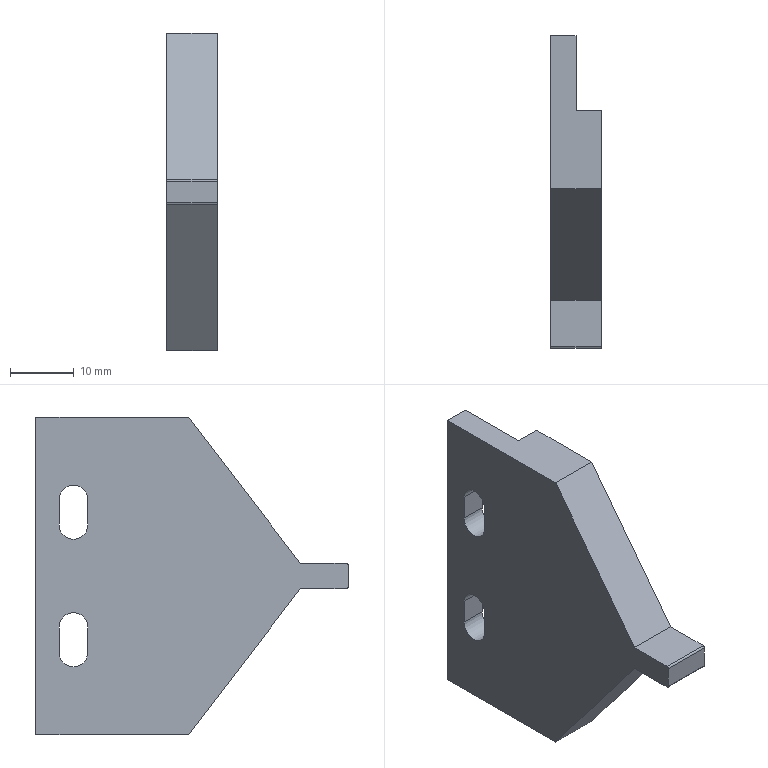Component | SolidWorks | WirePressingUnitPressingHead-2 | 1 solid | 24 faces | box 8 x 49 x 49.8 mm | volume 10945 mm3 | plane 16 | cylinder 8 | commonest cylinder face diameters 4.5 x6 0.6 x2
build123d program:
from build123d import *

# Parameters (mm, degrees)
BOSS_EXTRUDE1_DEPTH = 8
SKETCH2_W           = 49.8
SKETCH2_H           = 11.8
CUT_EXTRUDE1_DEPTH  = 4
SKETCH4_W           = 45.507
SKETCH4_H           = 8.951
BOSS_EXTRUDE2_DEPTH = 4
CUT_EXTRUDE3_DEPTH  = 10
FILLET1_R           = 0.3


with BuildPart() as part:
    # Sketch1 → Boss-Extrude1 (new body)
    with BuildSketch(Plane.XY):
        Polygon((2, 0), (2, 7.5), (24.9, 25), (24.9, 49), (-24.9, 49), (-24.9, 25), (-2, 7.5), (-2, 0), align=None)
    extrude(amount=BOSS_EXTRUDE1_DEPTH)

    # Sketch2 → Cut-Extrude1 (cut)
    with BuildSketch(Plane.XY.offset(8)):
        with Locations((0, 43.1)):
            Rectangle(SKETCH2_W, SKETCH2_H)
    extrude(amount=-CUT_EXTRUDE1_DEPTH, mode=Mode.SUBTRACT)

    # Sketch4 → Boss-Extrude2 (add)
    with BuildSketch(Plane(origin=(0, 0, 0), x_dir=(-1, 0, 0), z_dir=(0, 0, -1))):
        with Locations((-0.1161, 35.176)):
            Rectangle(SKETCH4_W, SKETCH4_H)
    extrude(amount=-BOSS_EXTRUDE2_DEPTH)

    # Sketch5 → Cut-Extrude3 (cut)
    with BuildSketch(Plane(origin=(0, 0, 0), x_dir=(-1, 0, 0), z_dir=(0, 0, -1))):
        with BuildLine():
            Line((-8, 40.85), (-12, 40.85))
            ThreePointArc((-12, 40.85), (-14.25, 43.1), (-12, 45.35))
            Line((-12, 45.35), (-8, 45.35))
            ThreePointArc((-8, 45.35), (-5.75, 43.1), (-8, 40.85))
        make_face()
        with BuildLine():
            Line((8, 45.35), (12, 45.35))
            ThreePointArc((12, 45.35), (14.25, 43.1), (12, 40.85))
            Line((12, 40.85), (8, 40.85))
            ThreePointArc((8, 40.85), (5.75, 43.1), (8, 45.35))
        make_face()
    extrude(amount=-CUT_EXTRUDE3_DEPTH, mode=Mode.SUBTRACT)

    # Fillet1
    fillet1_edges = [part.edges().sort_by_distance(p)[0] for p in [
        (-2, 0, 4),
        (2, 0, 4),
    ]]
    fillet(fillet1_edges, radius=FILLET1_R)


solid = part.part

# Placed as in the assembly
solid = solid.moved(Location((-17.235, -9.832, -145.015), (0, 90, 0)))
STEP:
#1=COLOUR_RGB('',0.7922,0.8196,0.9333);
#2=FILL_AREA_STYLE_COLOUR('',#1);
#3=FILL_AREA_STYLE('',(#2));
#4=SURFACE_STYLE_FILL_AREA(#3);
#5=SURFACE_SIDE_STYLE('',(#4));
#6=SURFACE_STYLE_USAGE(.BOTH.,#5);
#7=PRESENTATION_STYLE_ASSIGNMENT((#6));
#8=CARTESIAN_POINT('',(-0.5211,1.398,-5.237));
#9=VERTEX_POINT('',#8);
#10=CARTESIAN_POINT('',(-0.5211,1.31,-5.148));
#11=VERTEX_POINT('',#10);
#12=CARTESIAN_POINT('',(-0.5211,1.31,-5.237));
#13=DIRECTION('',(1.,0.,-0.));
#14=DIRECTION('',(-0.,0.,-1.));
#15=AXIS2_PLACEMENT_3D('',#12,#13,#14);
#16=CIRCLE('',#15,0.08858);
#17=EDGE_CURVE('',#9,#11,#16,.T.);
#18=ORIENTED_EDGE('',*,*,#17,.T.);
#19=CARTESIAN_POINT('',(-0.6786,1.31,-5.148));
#20=VERTEX_POINT('',#19);
#21=CARTESIAN_POINT('',(-0.2848,1.31,-5.148));
#22=DIRECTION('',(-1.,-0.,0.));
#23=VECTOR('',#22,39.37);
#24=LINE('',#21,#23);
#25=EDGE_CURVE('',#11,#20,#24,.T.);
#26=ORIENTED_EDGE('',*,*,#25,.T.);
#27=CARTESIAN_POINT('',(-0.6786,1.398,-5.237));
#28=VERTEX_POINT('',#27);
#29=CARTESIAN_POINT('',(-0.6786,1.31,-5.237));
#30=DIRECTION('',(-1.,-0.,0.));
#31=DIRECTION('',(0.,0.,1.));
#32=AXIS2_PLACEMENT_3D('',#29,#30,#31);
#33=CIRCLE('',#32,0.08858);
#34=EDGE_CURVE('',#20,#28,#33,.T.);
#35=ORIENTED_EDGE('',*,*,#34,.T.);
#36=CARTESIAN_POINT('',(-0.2848,1.398,-5.237));
#37=DIRECTION('',(-1.,-0.,0.));
#38=VECTOR('',#37,39.37);
#39=LINE('',#36,#38);
#40=EDGE_CURVE('',#9,#28,#39,.T.);
#41=ORIENTED_EDGE('',*,*,#40,.F.);
#42=EDGE_LOOP('',(#18,#26,#35,#41));
#43=FACE_OUTER_BOUND('',#42,.T.);
#44=CARTESIAN_POINT('',(-0.2848,1.31,-5.237));
#45=DIRECTION('',(-1.,-0.,0.));
#46=DIRECTION('',(0.,0.,1.));
#47=AXIS2_PLACEMENT_3D('',#44,#45,#46);
#48=CYLINDRICAL_SURFACE('',#47,0.08858);
#49=ADVANCED_FACE('',(#43),#48,.F.);
#50=CARTESIAN_POINT('',(-0.5211,1.398,-6.024));
#51=VERTEX_POINT('',#50);
#52=CARTESIAN_POINT('',(-0.5211,1.31,-5.936));
#53=VERTEX_POINT('',#52);
#54=CARTESIAN_POINT('',(-0.5211,1.31,-6.024));
#55=DIRECTION('',(1.,0.,-0.));
#56=DIRECTION('',(-0.,0.,-1.));
#57=AXIS2_PLACEMENT_3D('',#54,#55,#56);
#58=CIRCLE('',#57,0.08858);
#59=EDGE_CURVE('',#51,#53,#58,.T.);
#60=ORIENTED_EDGE('',*,*,#59,.T.);
#61=CARTESIAN_POINT('',(-0.6786,1.31,-5.936));
#62=VERTEX_POINT('',#61);
#63=CARTESIAN_POINT('',(-0.2848,1.31,-5.936));
#64=DIRECTION('',(-1.,-0.,0.));
#65=VECTOR('',#64,39.37);
#66=LINE('',#63,#65);
#67=EDGE_CURVE('',#53,#62,#66,.T.);
#68=ORIENTED_EDGE('',*,*,#67,.T.);
#69=CARTESIAN_POINT('',(-0.6786,1.398,-6.024));
#70=VERTEX_POINT('',#69);
#71=CARTESIAN_POINT('',(-0.6786,1.31,-6.024));
#72=DIRECTION('',(-1.,-0.,0.));
#73=DIRECTION('',(0.,0.,1.));
#74=AXIS2_PLACEMENT_3D('',#71,#72,#73);
#75=CIRCLE('',#74,0.08858);
#76=EDGE_CURVE('',#62,#70,#75,.T.);
#77=ORIENTED_EDGE('',*,*,#76,.T.);
#78=CARTESIAN_POINT('',(-0.2848,1.398,-6.024));
#79=DIRECTION('',(-1.,-0.,0.));
#80=VECTOR('',#79,39.37);
#81=LINE('',#78,#80);
#82=EDGE_CURVE('',#51,#70,#81,.T.);
#83=ORIENTED_EDGE('',*,*,#82,.F.);
#84=EDGE_LOOP('',(#60,#68,#77,#83));
#85=FACE_OUTER_BOUND('',#84,.T.);
#86=CARTESIAN_POINT('',(-0.2848,1.31,-6.024));
#87=DIRECTION('',(-1.,-0.,0.));
#88=DIRECTION('',(0.,0.,1.));
#89=AXIS2_PLACEMENT_3D('',#86,#87,#88);
#90=CYLINDRICAL_SURFACE('',#89,0.08858);
#91=ADVANCED_FACE('',(#85),#90,.F.);
#92=CARTESIAN_POINT('',(-0.5211,1.542,-6.69));
#93=VERTEX_POINT('',#92);
#94=CARTESIAN_POINT('',(-0.5211,1.542,-4.729));
#95=VERTEX_POINT('',#94);
#96=CARTESIAN_POINT('',(-0.5211,1.542,-4.729));
#97=DIRECTION('',(0.,-0.,1.));
#98=VECTOR('',#97,39.37);
#99=LINE('',#96,#98);
#100=EDGE_CURVE('',#93,#95,#99,.T.);
#101=ORIENTED_EDGE('',*,*,#100,.F.);
#102=CARTESIAN_POINT('',(-0.6786,1.542,-6.69));
#103=VERTEX_POINT('',#102);
#104=CARTESIAN_POINT('',(-0.3636,1.542,-6.69));
#105=DIRECTION('',(-1.,-0.,0.));
#106=VECTOR('',#105,39.37);
#107=LINE('',#104,#106);
#108=EDGE_CURVE('',#93,#103,#107,.T.);
#109=ORIENTED_EDGE('',*,*,#108,.T.);
#110=CARTESIAN_POINT('',(-0.6786,1.542,-4.729));
#111=VERTEX_POINT('',#110);
#112=CARTESIAN_POINT('',(-0.6786,1.542,-6.69));
#113=DIRECTION('',(0.,-0.,1.));
#114=VECTOR('',#113,39.37);
#115=LINE('',#112,#114);
#116=EDGE_CURVE('',#103,#111,#115,.T.);
#117=ORIENTED_EDGE('',*,*,#116,.T.);
#118=CARTESIAN_POINT('',(-0.3636,1.542,-4.729));
#119=DIRECTION('',(-1.,-0.,0.));
#120=VECTOR('',#119,39.37);
#121=LINE('',#118,#120);
#122=EDGE_CURVE('',#95,#111,#121,.T.);
#123=ORIENTED_EDGE('',*,*,#122,.F.);
#124=EDGE_LOOP('',(#101,#109,#117,#123));
#125=FACE_OUTER_BOUND('',#124,.T.);
#126=CARTESIAN_POINT('',(-0.3636,1.542,-6.69));
#127=DIRECTION('',(0.,-1.,-0.));
#128=DIRECTION('',(-1.,-0.,0.));
#129=AXIS2_PLACEMENT_3D('',#126,#127,#128);
#130=PLANE('',#129);
#131=ADVANCED_FACE('',(#125),#130,.F.);
#132=CARTESIAN_POINT('',(-0.6786,-0.3871,-5.642));
#133=VERTEX_POINT('',#132);
#134=CARTESIAN_POINT('',(-0.6786,-0.3871,-5.776));
#135=VERTEX_POINT('',#134);
#136=CARTESIAN_POINT('',(-0.6786,-0.3871,-5.631));
#137=DIRECTION('',(-0.,0.,-1.));
#138=VECTOR('',#137,39.37);
#139=LINE('',#136,#138);
#140=EDGE_CURVE('',#133,#135,#139,.T.);
#141=ORIENTED_EDGE('',*,*,#140,.T.);
#142=CARTESIAN_POINT('',(-0.3636,-0.3871,-5.776));
#143=VERTEX_POINT('',#142);
#144=CARTESIAN_POINT('',(-0.3636,-0.3871,-5.776));
#145=DIRECTION('',(1.,0.,-0.));
#146=VECTOR('',#145,39.37);
#147=LINE('',#144,#146);
#148=EDGE_CURVE('',#135,#143,#147,.T.);
#149=ORIENTED_EDGE('',*,*,#148,.T.);
#150=CARTESIAN_POINT('',(-0.3636,-0.3871,-5.642));
#151=VERTEX_POINT('',#150);
#152=CARTESIAN_POINT('',(-0.3636,-0.3871,-5.631));
#153=DIRECTION('',(-0.,0.,-1.));
#154=VECTOR('',#153,39.37);
#155=LINE('',#152,#154);
#156=EDGE_CURVE('',#151,#143,#155,.T.);
#157=ORIENTED_EDGE('',*,*,#156,.F.);
#158=CARTESIAN_POINT('',(-0.3636,-0.3871,-5.642));
#159=DIRECTION('',(-1.,-0.,0.));
#160=VECTOR('',#159,39.37);
#161=LINE('',#158,#160);
#162=EDGE_CURVE('',#151,#133,#161,.T.);
#163=ORIENTED_EDGE('',*,*,#162,.T.);
#164=EDGE_LOOP('',(#141,#149,#157,#163));
#165=FACE_OUTER_BOUND('',#164,.T.);
#166=CARTESIAN_POINT('',(-0.3636,-0.3871,-5.631));
#167=DIRECTION('',(-0.,1.,0.));
#168=DIRECTION('',(1.,0.,-0.));
#169=AXIS2_PLACEMENT_3D('',#166,#167,#168);
#170=PLANE('',#169);
#171=ADVANCED_FACE('',(#165),#170,.F.);
#172=CARTESIAN_POINT('',(-0.3636,-0.3753,-5.788));
#173=VERTEX_POINT('',#172);
#174=CARTESIAN_POINT('',(-0.3636,-0.0918,-5.788));
#175=VERTEX_POINT('',#174);
#176=CARTESIAN_POINT('',(-0.3636,-0.3871,-5.788));
#177=DIRECTION('',(-0.,1.,0.));
#178=VECTOR('',#177,39.37);
#179=LINE('',#176,#178);
#180=EDGE_CURVE('',#173,#175,#179,.T.);
#181=ORIENTED_EDGE('',*,*,#180,.F.);
#182=CARTESIAN_POINT('',(-0.6786,-0.3753,-5.788));
#183=VERTEX_POINT('',#182);
#184=CARTESIAN_POINT('',(-0.3636,-0.3753,-5.788));
#185=DIRECTION('',(-1.,-0.,0.));
#186=VECTOR('',#185,39.37);
#187=LINE('',#184,#186);
#188=EDGE_CURVE('',#173,#183,#187,.T.);
#189=ORIENTED_EDGE('',*,*,#188,.T.);
#190=CARTESIAN_POINT('',(-0.6786,-0.0918,-5.788));
#191=VERTEX_POINT('',#190);
#192=CARTESIAN_POINT('',(-0.6786,-0.3871,-5.788));
#193=DIRECTION('',(-0.,1.,0.));
#194=VECTOR('',#193,39.37);
#195=LINE('',#192,#194);
#196=EDGE_CURVE('',#183,#191,#195,.T.);
#197=ORIENTED_EDGE('',*,*,#196,.T.);
#198=CARTESIAN_POINT('',(-0.3636,-0.0918,-5.788));
#199=DIRECTION('',(-1.,-0.,0.));
#200=VECTOR('',#199,39.37);
#201=LINE('',#198,#200);
#202=EDGE_CURVE('',#175,#191,#201,.T.);
#203=ORIENTED_EDGE('',*,*,#202,.F.);
#204=EDGE_LOOP('',(#181,#189,#197,#203));
#205=FACE_OUTER_BOUND('',#204,.T.);
#206=CARTESIAN_POINT('',(-0.3636,-0.3871,-5.788));
#207=DIRECTION('',(0.,-0.,1.));
#208=DIRECTION('',(1.,0.,-0.));
#209=AXIS2_PLACEMENT_3D('',#206,#207,#208);
#210=PLANE('',#209);
#211=ADVANCED_FACE('',(#205),#210,.F.);
#212=CARTESIAN_POINT('',(-0.6786,0.5972,-6.69));
#213=VERTEX_POINT('',#212);
#214=CARTESIAN_POINT('',(-0.6786,-0.0918,-5.788));
#215=DIRECTION('',(-0.,0.6072,-0.7946));
#216=VECTOR('',#215,39.37);
#217=LINE('',#214,#216);
#218=EDGE_CURVE('',#191,#213,#217,.T.);
#219=ORIENTED_EDGE('',*,*,#218,.T.);
#220=CARTESIAN_POINT('',(-0.3636,0.5972,-6.69));
#221=VERTEX_POINT('',#220);
#222=CARTESIAN_POINT('',(-0.3636,0.5972,-6.69));
#223=DIRECTION('',(-1.,-0.,0.));
#224=VECTOR('',#223,39.37);
#225=LINE('',#222,#224);
#226=EDGE_CURVE('',#221,#213,#225,.T.);
#227=ORIENTED_EDGE('',*,*,#226,.F.);
#228=CARTESIAN_POINT('',(-0.3636,-0.0918,-5.788));
#229=DIRECTION('',(-0.,0.6072,-0.7946));
#230=VECTOR('',#229,39.37);
#231=LINE('',#228,#230);
#232=EDGE_CURVE('',#175,#221,#231,.T.);
#233=ORIENTED_EDGE('',*,*,#232,.F.);
#234=ORIENTED_EDGE('',*,*,#202,.T.);
#235=EDGE_LOOP('',(#219,#227,#233,#234));
#236=FACE_OUTER_BOUND('',#235,.T.);
#237=CARTESIAN_POINT('',(-0.3636,-0.0918,-5.788));
#238=DIRECTION('',(0.,0.7946,0.6072));
#239=DIRECTION('',(0.,-0.6072,0.7946));
#240=AXIS2_PLACEMENT_3D('',#237,#238,#239);
#241=PLANE('',#240);
#242=ADVANCED_FACE('',(#236),#241,.F.);
#243=CARTESIAN_POINT('',(-0.5211,1.077,-6.69));
#244=VERTEX_POINT('',#243);
#245=CARTESIAN_POINT('',(-0.5211,1.542,-6.69));
#246=DIRECTION('',(-0.,1.,0.));
#247=VECTOR('',#246,39.37);
#248=LINE('',#245,#247);
#249=EDGE_CURVE('',#244,#93,#248,.T.);
#250=ORIENTED_EDGE('',*,*,#249,.F.);
#251=CARTESIAN_POINT('',(-0.3636,1.077,-6.69));
#252=VERTEX_POINT('',#251);
#253=CARTESIAN_POINT('',(-0.5211,1.077,-6.69));
#254=DIRECTION('',(1.,0.,-0.));
#255=VECTOR('',#254,39.37);
#256=LINE('',#253,#255);
#257=EDGE_CURVE('',#244,#252,#256,.T.);
#258=ORIENTED_EDGE('',*,*,#257,.T.);
#259=CARTESIAN_POINT('',(-0.3636,0.5972,-6.69));
#260=DIRECTION('',(-0.,1.,0.));
#261=VECTOR('',#260,39.37);
#262=LINE('',#259,#261);
#263=EDGE_CURVE('',#221,#252,#262,.T.);
#264=ORIENTED_EDGE('',*,*,#263,.F.);
#265=ORIENTED_EDGE('',*,*,#226,.T.);
#266=CARTESIAN_POINT('',(-0.6786,0.5972,-6.69));
#267=DIRECTION('',(-0.,1.,0.));
#268=VECTOR('',#267,39.37);
#269=LINE('',#266,#268);
#270=EDGE_CURVE('',#213,#103,#269,.T.);
#271=ORIENTED_EDGE('',*,*,#270,.T.);
#272=ORIENTED_EDGE('',*,*,#108,.F.);
#273=EDGE_LOOP('',(#250,#258,#264,#265,#271,#272));
#274=FACE_OUTER_BOUND('',#273,.T.);
#275=CARTESIAN_POINT('',(-0.3636,0.5972,-6.69));
#276=DIRECTION('',(0.,-0.,1.));
#277=DIRECTION('',(1.,0.,-0.));
#278=AXIS2_PLACEMENT_3D('',#275,#276,#277);
#279=PLANE('',#278);
#280=ADVANCED_FACE('',(#274),#279,.F.);
#281=CARTESIAN_POINT('',(-0.3636,1.077,-4.729));
#282=VERTEX_POINT('',#281);
#283=CARTESIAN_POINT('',(-0.3636,0.5972,-4.729));
#284=VERTEX_POINT('',#283);
#285=CARTESIAN_POINT('',(-0.3636,0.5972,-4.729));
#286=DIRECTION('',(0.,-1.,-0.));
#287=VECTOR('',#286,39.37);
#288=LINE('',#285,#287);
#289=EDGE_CURVE('',#282,#284,#288,.T.);
#290=ORIENTED_EDGE('',*,*,#289,.F.);
#291=CARTESIAN_POINT('',(-0.5211,1.077,-4.729));
#292=VERTEX_POINT('',#291);
#293=CARTESIAN_POINT('',(-0.5211,1.077,-4.729));
#294=DIRECTION('',(1.,0.,-0.));
#295=VECTOR('',#294,39.37);
#296=LINE('',#293,#295);
#297=EDGE_CURVE('',#292,#282,#296,.T.);
#298=ORIENTED_EDGE('',*,*,#297,.F.);
#299=CARTESIAN_POINT('',(-0.5211,1.542,-4.729));
#300=DIRECTION('',(0.,-1.,-0.));
#301=VECTOR('',#300,39.37);
#302=LINE('',#299,#301);
#303=EDGE_CURVE('',#95,#292,#302,.T.);
#304=ORIENTED_EDGE('',*,*,#303,.F.);
#305=ORIENTED_EDGE('',*,*,#122,.T.);
#306=CARTESIAN_POINT('',(-0.6786,0.5972,-4.729));
#307=VERTEX_POINT('',#306);
#308=CARTESIAN_POINT('',(-0.6786,0.5972,-4.729));
#309=DIRECTION('',(0.,-1.,-0.));
#310=VECTOR('',#309,39.37);
#311=LINE('',#308,#310);
#312=EDGE_CURVE('',#111,#307,#311,.T.);
#313=ORIENTED_EDGE('',*,*,#312,.T.);
#314=CARTESIAN_POINT('',(-0.3636,0.5972,-4.729));
#315=DIRECTION('',(-1.,-0.,0.));
#316=VECTOR('',#315,39.37);
#317=LINE('',#314,#316);
#318=EDGE_CURVE('',#284,#307,#317,.T.);
#319=ORIENTED_EDGE('',*,*,#318,.F.);
#320=EDGE_LOOP('',(#290,#298,#304,#305,#313,#319));
#321=FACE_OUTER_BOUND('',#320,.T.);
#322=CARTESIAN_POINT('',(-0.3636,0.5972,-4.729));
#323=DIRECTION('',(-0.,0.,-1.));
#324=DIRECTION('',(-1.,-0.,0.));
#325=AXIS2_PLACEMENT_3D('',#322,#323,#324);
#326=PLANE('',#325);
#327=ADVANCED_FACE('',(#321),#326,.F.);
#328=CARTESIAN_POINT('',(-0.6786,-0.0918,-5.631));
#329=VERTEX_POINT('',#328);
#330=CARTESIAN_POINT('',(-0.6786,-0.0918,-5.631));
#331=DIRECTION('',(-0.,-0.6072,-0.7946));
#332=VECTOR('',#331,39.37);
#333=LINE('',#330,#332);
#334=EDGE_CURVE('',#307,#329,#333,.T.);
#335=ORIENTED_EDGE('',*,*,#334,.T.);
#336=CARTESIAN_POINT('',(-0.3636,-0.0918,-5.631));
#337=VERTEX_POINT('',#336);
#338=CARTESIAN_POINT('',(-0.3636,-0.0918,-5.631));
#339=DIRECTION('',(-1.,-0.,0.));
#340=VECTOR('',#339,39.37);
#341=LINE('',#338,#340);
#342=EDGE_CURVE('',#337,#329,#341,.T.);
#343=ORIENTED_EDGE('',*,*,#342,.F.);
#344=CARTESIAN_POINT('',(-0.3636,-0.0918,-5.631));
#345=DIRECTION('',(-0.,-0.6072,-0.7946));
#346=VECTOR('',#345,39.37);
#347=LINE('',#344,#346);
#348=EDGE_CURVE('',#284,#337,#347,.T.);
#349=ORIENTED_EDGE('',*,*,#348,.F.);
#350=ORIENTED_EDGE('',*,*,#318,.T.);
#351=EDGE_LOOP('',(#335,#343,#349,#350));
#352=FACE_OUTER_BOUND('',#351,.T.);
#353=CARTESIAN_POINT('',(-0.3636,-0.0918,-5.631));
#354=DIRECTION('',(-0.,0.7946,-0.6072));
#355=DIRECTION('',(0.,0.6072,0.7946));
#356=AXIS2_PLACEMENT_3D('',#353,#354,#355);
#357=PLANE('',#356);
#358=ADVANCED_FACE('',(#352),#357,.F.);
#359=CARTESIAN_POINT('',(-0.6786,-0.3753,-5.631));
#360=VERTEX_POINT('',#359);
#361=CARTESIAN_POINT('',(-0.6786,-0.3871,-5.631));
#362=DIRECTION('',(0.,-1.,-0.));
#363=VECTOR('',#362,39.37);
#364=LINE('',#361,#363);
#365=EDGE_CURVE('',#329,#360,#364,.T.);
#366=ORIENTED_EDGE('',*,*,#365,.T.);
#367=CARTESIAN_POINT('',(-0.3636,-0.3753,-5.631));
#368=VERTEX_POINT('',#367);
#369=CARTESIAN_POINT('',(-0.3636,-0.3753,-5.631));
#370=DIRECTION('',(1.,0.,-0.));
#371=VECTOR('',#370,39.37);
#372=LINE('',#369,#371);
#373=EDGE_CURVE('',#360,#368,#372,.T.);
#374=ORIENTED_EDGE('',*,*,#373,.T.);
#375=CARTESIAN_POINT('',(-0.3636,-0.3871,-5.631));
#376=DIRECTION('',(0.,-1.,-0.));
#377=VECTOR('',#376,39.37);
#378=LINE('',#375,#377);
#379=EDGE_CURVE('',#337,#368,#378,.T.);
#380=ORIENTED_EDGE('',*,*,#379,.F.);
#381=ORIENTED_EDGE('',*,*,#342,.T.);
#382=EDGE_LOOP('',(#366,#374,#380,#381));
#383=FACE_OUTER_BOUND('',#382,.T.);
#384=CARTESIAN_POINT('',(-0.3636,-0.3871,-5.631));
#385=DIRECTION('',(-0.,0.,-1.));
#386=DIRECTION('',(-1.,-0.,0.));
#387=AXIS2_PLACEMENT_3D('',#384,#385,#386);
#388=PLANE('',#387);
#389=ADVANCED_FACE('',(#383),#388,.F.);
#390=ORIENTED_EDGE('',*,*,#156,.T.);
#391=CARTESIAN_POINT('',(-0.3636,-0.3753,-5.776));
#392=DIRECTION('',(1.,0.,-0.));
#393=DIRECTION('',(0.,0.,-1.));
#394=AXIS2_PLACEMENT_3D('',#391,#392,#393);
#395=CIRCLE('',#394,0.01181);
#396=EDGE_CURVE('',#143,#173,#395,.T.);
#397=ORIENTED_EDGE('',*,*,#396,.T.);
#398=ORIENTED_EDGE('',*,*,#180,.T.);
#399=ORIENTED_EDGE('',*,*,#232,.T.);
#400=ORIENTED_EDGE('',*,*,#263,.T.);
#401=CARTESIAN_POINT('',(-0.3636,1.077,-4.729));
#402=DIRECTION('',(-0.,0.,-1.));
#403=VECTOR('',#402,39.37);
#404=LINE('',#401,#403);
#405=EDGE_CURVE('',#282,#252,#404,.T.);
#406=ORIENTED_EDGE('',*,*,#405,.F.);
#407=ORIENTED_EDGE('',*,*,#289,.T.);
#408=ORIENTED_EDGE('',*,*,#348,.T.);
#409=ORIENTED_EDGE('',*,*,#379,.T.);
#410=CARTESIAN_POINT('',(-0.3636,-0.3753,-5.642));
#411=DIRECTION('',(1.,0.,-0.));
#412=DIRECTION('',(0.,0.,-1.));
#413=AXIS2_PLACEMENT_3D('',#410,#411,#412);
#414=CIRCLE('',#413,0.01181);
#415=EDGE_CURVE('',#368,#151,#414,.T.);
#416=ORIENTED_EDGE('',*,*,#415,.T.);
#417=EDGE_LOOP('',(#390,#397,#398,#399,#400,#406,#407,#408,#409,#416));
#418=FACE_OUTER_BOUND('',#417,.T.);
#419=CARTESIAN_POINT('',(-0.3636,-0.3871,-5.788));
#420=DIRECTION('',(1.,0.,-0.));
#421=DIRECTION('',(-0.,0.,-1.));
#422=AXIS2_PLACEMENT_3D('',#419,#420,#421);
#423=PLANE('',#422);
#424=ADVANCED_FACE('',(#418),#423,.T.);
#425=CARTESIAN_POINT('',(-0.6786,1.221,-5.394));
#426=VERTEX_POINT('',#425);
#427=CARTESIAN_POINT('',(-0.6786,1.221,-5.237));
#428=VERTEX_POINT('',#427);
#429=CARTESIAN_POINT('',(-0.6786,1.221,-5.394));
#430=DIRECTION('',(0.,-0.,1.));
#431=VECTOR('',#430,39.37);
#432=LINE('',#429,#431);
#433=EDGE_CURVE('',#426,#428,#432,.T.);
#434=ORIENTED_EDGE('',*,*,#433,.F.);
#435=CARTESIAN_POINT('',(-0.6786,1.398,-5.394));
#436=VERTEX_POINT('',#435);
#437=CARTESIAN_POINT('',(-0.6786,1.31,-5.394));
#438=DIRECTION('',(-1.,-0.,0.));
#439=DIRECTION('',(0.,0.,1.));
#440=AXIS2_PLACEMENT_3D('',#437,#438,#439);
#441=CIRCLE('',#440,0.08858);
#442=EDGE_CURVE('',#436,#426,#441,.T.);
#443=ORIENTED_EDGE('',*,*,#442,.F.);
#444=CARTESIAN_POINT('',(-0.6786,1.398,-5.394));
#445=DIRECTION('',(-0.,0.,-1.));
#446=VECTOR('',#445,39.37);
#447=LINE('',#444,#446);
#448=EDGE_CURVE('',#28,#436,#447,.T.);
#449=ORIENTED_EDGE('',*,*,#448,.F.);
#450=ORIENTED_EDGE('',*,*,#34,.F.);
#451=CARTESIAN_POINT('',(-0.6786,1.31,-5.237));
#452=DIRECTION('',(-1.,-0.,0.));
#453=DIRECTION('',(0.,0.,1.));
#454=AXIS2_PLACEMENT_3D('',#451,#452,#453);
#455=CIRCLE('',#454,0.08858);
#456=EDGE_CURVE('',#428,#20,#455,.T.);
#457=ORIENTED_EDGE('',*,*,#456,.F.);
#458=EDGE_LOOP('',(#434,#443,#449,#450,#457));
#459=FACE_BOUND('',#458,.T.);
#460=CARTESIAN_POINT('',(-0.6786,1.398,-6.182));
#461=VERTEX_POINT('',#460);
#462=CARTESIAN_POINT('',(-0.6786,1.398,-6.024));
#463=DIRECTION('',(-0.,0.,-1.));
#464=VECTOR('',#463,39.37);
#465=LINE('',#462,#464);
#466=EDGE_CURVE('',#70,#461,#465,.T.);
#467=ORIENTED_EDGE('',*,*,#466,.F.);
#468=ORIENTED_EDGE('',*,*,#76,.F.);
#469=CARTESIAN_POINT('',(-0.6786,1.221,-6.024));
#470=VERTEX_POINT('',#469);
#471=CARTESIAN_POINT('',(-0.6786,1.31,-6.024));
#472=DIRECTION('',(-1.,-0.,0.));
#473=DIRECTION('',(0.,0.,1.));
#474=AXIS2_PLACEMENT_3D('',#471,#472,#473);
#475=CIRCLE('',#474,0.08858);
#476=EDGE_CURVE('',#470,#62,#475,.T.);
#477=ORIENTED_EDGE('',*,*,#476,.F.);
#478=CARTESIAN_POINT('',(-0.6786,1.221,-6.182));
#479=VERTEX_POINT('',#478);
#480=CARTESIAN_POINT('',(-0.6786,1.221,-6.024));
#481=DIRECTION('',(0.,-0.,1.));
#482=VECTOR('',#481,39.37);
#483=LINE('',#480,#482);
#484=EDGE_CURVE('',#479,#470,#483,.T.);
#485=ORIENTED_EDGE('',*,*,#484,.F.);
#486=CARTESIAN_POINT('',(-0.6786,1.31,-6.182));
#487=DIRECTION('',(-1.,-0.,0.));
#488=DIRECTION('',(0.,0.,1.));
#489=AXIS2_PLACEMENT_3D('',#486,#487,#488);
#490=CIRCLE('',#489,0.08858);
#491=EDGE_CURVE('',#461,#479,#490,.T.);
#492=ORIENTED_EDGE('',*,*,#491,.F.);
#493=EDGE_LOOP('',(#467,#468,#477,#485,#492));
#494=FACE_BOUND('',#493,.T.);
#495=ORIENTED_EDGE('',*,*,#196,.F.);
#496=CARTESIAN_POINT('',(-0.6786,-0.3753,-5.776));
#497=DIRECTION('',(-1.,-0.,0.));
#498=DIRECTION('',(0.,0.,-1.));
#499=AXIS2_PLACEMENT_3D('',#496,#497,#498);
#500=CIRCLE('',#499,0.01181);
#501=EDGE_CURVE('',#183,#135,#500,.T.);
#502=ORIENTED_EDGE('',*,*,#501,.T.);
#503=ORIENTED_EDGE('',*,*,#140,.F.);
#504=CARTESIAN_POINT('',(-0.6786,-0.3753,-5.642));
#505=DIRECTION('',(-1.,-0.,0.));
#506=DIRECTION('',(0.,0.,-1.));
#507=AXIS2_PLACEMENT_3D('',#504,#505,#506);
#508=CIRCLE('',#507,0.01181);
#509=EDGE_CURVE('',#133,#360,#508,.T.);
#510=ORIENTED_EDGE('',*,*,#509,.T.);
#511=ORIENTED_EDGE('',*,*,#365,.F.);
#512=ORIENTED_EDGE('',*,*,#334,.F.);
#513=ORIENTED_EDGE('',*,*,#312,.F.);
#514=ORIENTED_EDGE('',*,*,#116,.F.);
#515=ORIENTED_EDGE('',*,*,#270,.F.);
#516=ORIENTED_EDGE('',*,*,#218,.F.);
#517=EDGE_LOOP('',(#495,#502,#503,#510,#511,#512,#513,#514,#515,#516));
#518=FACE_OUTER_BOUND('',#517,.T.);
#519=CARTESIAN_POINT('',(-0.6786,-0.3871,-5.788));
#520=DIRECTION('',(1.,0.,-0.));
#521=DIRECTION('',(-0.,0.,-1.));
#522=AXIS2_PLACEMENT_3D('',#519,#520,#521);
#523=PLANE('',#522);
#524=ADVANCED_FACE('',(#459,#494,#518),#523,.F.);
#525=ORIENTED_EDGE('',*,*,#405,.T.);
#526=ORIENTED_EDGE('',*,*,#257,.F.);
#527=CARTESIAN_POINT('',(-0.5211,1.077,-4.729));
#528=DIRECTION('',(-0.,0.,-1.));
#529=VECTOR('',#528,39.37);
#530=LINE('',#527,#529);
#531=EDGE_CURVE('',#292,#244,#530,.T.);
#532=ORIENTED_EDGE('',*,*,#531,.F.);
#533=ORIENTED_EDGE('',*,*,#297,.T.);
#534=EDGE_LOOP('',(#525,#526,#532,#533));
#535=FACE_OUTER_BOUND('',#534,.T.);
#536=CARTESIAN_POINT('',(-0.5211,1.077,-4.729));
#537=DIRECTION('',(0.,-1.,-0.));
#538=DIRECTION('',(-1.,-0.,0.));
#539=AXIS2_PLACEMENT_3D('',#536,#537,#538);
#540=PLANE('',#539);
#541=ADVANCED_FACE('',(#535),#540,.F.);
#542=CARTESIAN_POINT('',(-0.5211,1.221,-5.394));
#543=VERTEX_POINT('',#542);
#544=CARTESIAN_POINT('',(-0.5211,1.398,-5.394));
#545=VERTEX_POINT('',#544);
#546=CARTESIAN_POINT('',(-0.5211,1.31,-5.394));
#547=DIRECTION('',(1.,0.,-0.));
#548=DIRECTION('',(-0.,0.,-1.));
#549=AXIS2_PLACEMENT_3D('',#546,#547,#548);
#550=CIRCLE('',#549,0.08858);
#551=EDGE_CURVE('',#543,#545,#550,.T.);
#552=ORIENTED_EDGE('',*,*,#551,.F.);
#553=CARTESIAN_POINT('',(-0.5211,1.221,-5.237));
#554=VERTEX_POINT('',#553);
#555=CARTESIAN_POINT('',(-0.5211,1.221,-4.729));
#556=DIRECTION('',(-0.,0.,-1.));
#557=VECTOR('',#556,39.37);
#558=LINE('',#555,#557);
#559=EDGE_CURVE('',#554,#543,#558,.T.);
#560=ORIENTED_EDGE('',*,*,#559,.F.);
#561=CARTESIAN_POINT('',(-0.5211,1.31,-5.237));
#562=DIRECTION('',(1.,0.,-0.));
#563=DIRECTION('',(-0.,0.,-1.));
#564=AXIS2_PLACEMENT_3D('',#561,#562,#563);
#565=CIRCLE('',#564,0.08858);
#566=EDGE_CURVE('',#11,#554,#565,.T.);
#567=ORIENTED_EDGE('',*,*,#566,.F.);
#568=ORIENTED_EDGE('',*,*,#17,.F.);
#569=CARTESIAN_POINT('',(-0.5211,1.398,-4.729));
#570=DIRECTION('',(0.,-0.,1.));
#571=VECTOR('',#570,39.37);
#572=LINE('',#569,#571);
#573=EDGE_CURVE('',#545,#9,#572,.T.);
#574=ORIENTED_EDGE('',*,*,#573,.F.);
#575=EDGE_LOOP('',(#552,#560,#567,#568,#574));
#576=FACE_BOUND('',#575,.T.);
#577=ORIENTED_EDGE('',*,*,#59,.F.);
#578=CARTESIAN_POINT('',(-0.5211,1.398,-6.182));
#579=VERTEX_POINT('',#578);
#580=CARTESIAN_POINT('',(-0.5211,1.398,-4.729));
#581=DIRECTION('',(0.,-0.,1.));
#582=VECTOR('',#581,39.37);
#583=LINE('',#580,#582);
#584=EDGE_CURVE('',#579,#51,#583,.T.);
#585=ORIENTED_EDGE('',*,*,#584,.F.);
#586=CARTESIAN_POINT('',(-0.5211,1.221,-6.182));
#587=VERTEX_POINT('',#586);
#588=CARTESIAN_POINT('',(-0.5211,1.31,-6.182));
#589=DIRECTION('',(1.,0.,-0.));
#590=DIRECTION('',(-0.,0.,-1.));
#591=AXIS2_PLACEMENT_3D('',#588,#589,#590);
#592=CIRCLE('',#591,0.08858);
#593=EDGE_CURVE('',#587,#579,#592,.T.);
#594=ORIENTED_EDGE('',*,*,#593,.F.);
#595=CARTESIAN_POINT('',(-0.5211,1.221,-6.024));
#596=VERTEX_POINT('',#595);
#597=CARTESIAN_POINT('',(-0.5211,1.221,-4.729));
#598=DIRECTION('',(-0.,0.,-1.));
#599=VECTOR('',#598,39.37);
#600=LINE('',#597,#599);
#601=EDGE_CURVE('',#596,#587,#600,.T.);
#602=ORIENTED_EDGE('',*,*,#601,.F.);
#603=CARTESIAN_POINT('',(-0.5211,1.31,-6.024));
#604=DIRECTION('',(1.,0.,-0.));
#605=DIRECTION('',(-0.,0.,-1.));
#606=AXIS2_PLACEMENT_3D('',#603,#604,#605);
#607=CIRCLE('',#606,0.08858);
#608=EDGE_CURVE('',#53,#596,#607,.T.);
#609=ORIENTED_EDGE('',*,*,#608,.F.);
#610=EDGE_LOOP('',(#577,#585,#594,#602,#609));
#611=FACE_BOUND('',#610,.T.);
#612=ORIENTED_EDGE('',*,*,#531,.T.);
#613=ORIENTED_EDGE('',*,*,#249,.T.);
#614=ORIENTED_EDGE('',*,*,#100,.T.);
#615=ORIENTED_EDGE('',*,*,#303,.T.);
#616=EDGE_LOOP('',(#612,#613,#614,#615));
#617=FACE_OUTER_BOUND('',#616,.T.);
#618=CARTESIAN_POINT('',(-0.5211,1.077,-4.729));
#619=DIRECTION('',(1.,0.,-0.));
#620=DIRECTION('',(-0.,0.,-1.));
#621=AXIS2_PLACEMENT_3D('',#618,#619,#620);
#622=PLANE('',#621);
#623=ADVANCED_FACE('',(#576,#611,#617),#622,.T.);
#624=ORIENTED_EDGE('',*,*,#67,.F.);
#625=ORIENTED_EDGE('',*,*,#608,.T.);
#626=CARTESIAN_POINT('',(-0.2848,1.221,-6.024));
#627=DIRECTION('',(-1.,-0.,0.));
#628=VECTOR('',#627,39.37);
#629=LINE('',#626,#628);
#630=EDGE_CURVE('',#596,#470,#629,.T.);
#631=ORIENTED_EDGE('',*,*,#630,.T.);
#632=ORIENTED_EDGE('',*,*,#476,.T.);
#633=EDGE_LOOP('',(#624,#625,#631,#632));
#634=FACE_OUTER_BOUND('',#633,.T.);
#635=CARTESIAN_POINT('',(-0.2848,1.31,-6.024));
#636=DIRECTION('',(-1.,-0.,0.));
#637=DIRECTION('',(0.,0.,1.));
#638=AXIS2_PLACEMENT_3D('',#635,#636,#637);
#639=CYLINDRICAL_SURFACE('',#638,0.08858);
#640=ADVANCED_FACE('',(#634),#639,.F.);
#641=ORIENTED_EDGE('',*,*,#601,.T.);
#642=CARTESIAN_POINT('',(-0.2848,1.221,-6.182));
#643=DIRECTION('',(-1.,-0.,0.));
#644=VECTOR('',#643,39.37);
#645=LINE('',#642,#644);
#646=EDGE_CURVE('',#587,#479,#645,.T.);
#647=ORIENTED_EDGE('',*,*,#646,.T.);
#648=ORIENTED_EDGE('',*,*,#484,.T.);
#649=ORIENTED_EDGE('',*,*,#630,.F.);
#650=EDGE_LOOP('',(#641,#647,#648,#649));
#651=FACE_OUTER_BOUND('',#650,.T.);
#652=CARTESIAN_POINT('',(-0.2848,1.221,-6.024));
#653=DIRECTION('',(0.,-1.,-0.));
#654=DIRECTION('',(-1.,-0.,0.));
#655=AXIS2_PLACEMENT_3D('',#652,#653,#654);
#656=PLANE('',#655);
#657=ADVANCED_FACE('',(#651),#656,.F.);
#658=ORIENTED_EDGE('',*,*,#593,.T.);
#659=CARTESIAN_POINT('',(-0.2848,1.398,-6.182));
#660=DIRECTION('',(-1.,-0.,0.));
#661=VECTOR('',#660,39.37);
#662=LINE('',#659,#661);
#663=EDGE_CURVE('',#579,#461,#662,.T.);
#664=ORIENTED_EDGE('',*,*,#663,.T.);
#665=ORIENTED_EDGE('',*,*,#491,.T.);
#666=ORIENTED_EDGE('',*,*,#646,.F.);
#667=EDGE_LOOP('',(#658,#664,#665,#666));
#668=FACE_OUTER_BOUND('',#667,.T.);
#669=CARTESIAN_POINT('',(-0.2848,1.31,-6.182));
#670=DIRECTION('',(-1.,-0.,0.));
#671=DIRECTION('',(0.,0.,1.));
#672=AXIS2_PLACEMENT_3D('',#669,#670,#671);
#673=CYLINDRICAL_SURFACE('',#672,0.08858);
#674=ADVANCED_FACE('',(#668),#673,.F.);
#675=ORIENTED_EDGE('',*,*,#584,.T.);
#676=ORIENTED_EDGE('',*,*,#82,.T.);
#677=ORIENTED_EDGE('',*,*,#466,.T.);
#678=ORIENTED_EDGE('',*,*,#663,.F.);
#679=EDGE_LOOP('',(#675,#676,#677,#678));
#680=FACE_OUTER_BOUND('',#679,.T.);
#681=CARTESIAN_POINT('',(-0.2848,1.398,-6.024));
#682=DIRECTION('',(-0.,1.,0.));
#683=DIRECTION('',(1.,0.,-0.));
#684=AXIS2_PLACEMENT_3D('',#681,#682,#683);
#685=PLANE('',#684);
#686=ADVANCED_FACE('',(#680),#685,.F.);
#687=ORIENTED_EDGE('',*,*,#551,.T.);
#688=CARTESIAN_POINT('',(-0.2848,1.398,-5.394));
#689=DIRECTION('',(-1.,-0.,0.));
#690=VECTOR('',#689,39.37);
#691=LINE('',#688,#690);
#692=EDGE_CURVE('',#545,#436,#691,.T.);
#693=ORIENTED_EDGE('',*,*,#692,.T.);
#694=ORIENTED_EDGE('',*,*,#442,.T.);
#695=CARTESIAN_POINT('',(-0.2848,1.221,-5.394));
#696=DIRECTION('',(-1.,-0.,0.));
#697=VECTOR('',#696,39.37);
#698=LINE('',#695,#697);
#699=EDGE_CURVE('',#543,#426,#698,.T.);
#700=ORIENTED_EDGE('',*,*,#699,.F.);
#701=EDGE_LOOP('',(#687,#693,#694,#700));
#702=FACE_OUTER_BOUND('',#701,.T.);
#703=CARTESIAN_POINT('',(-0.2848,1.31,-5.394));
#704=DIRECTION('',(-1.,-0.,0.));
#705=DIRECTION('',(0.,0.,1.));
#706=AXIS2_PLACEMENT_3D('',#703,#704,#705);
#707=CYLINDRICAL_SURFACE('',#706,0.08858);
#708=ADVANCED_FACE('',(#702),#707,.F.);
#709=ORIENTED_EDGE('',*,*,#573,.T.);
#710=ORIENTED_EDGE('',*,*,#40,.T.);
#711=ORIENTED_EDGE('',*,*,#448,.T.);
#712=ORIENTED_EDGE('',*,*,#692,.F.);
#713=EDGE_LOOP('',(#709,#710,#711,#712));
#714=FACE_OUTER_BOUND('',#713,.T.);
#715=CARTESIAN_POINT('',(-0.2848,1.398,-5.394));
#716=DIRECTION('',(-0.,1.,0.));
#717=DIRECTION('',(1.,0.,-0.));
#718=AXIS2_PLACEMENT_3D('',#715,#716,#717);
#719=PLANE('',#718);
#720=ADVANCED_FACE('',(#714),#719,.F.);
#721=ORIENTED_EDGE('',*,*,#25,.F.);
#722=ORIENTED_EDGE('',*,*,#566,.T.);
#723=CARTESIAN_POINT('',(-0.2848,1.221,-5.237));
#724=DIRECTION('',(-1.,-0.,0.));
#725=VECTOR('',#724,39.37);
#726=LINE('',#723,#725);
#727=EDGE_CURVE('',#554,#428,#726,.T.);
#728=ORIENTED_EDGE('',*,*,#727,.T.);
#729=ORIENTED_EDGE('',*,*,#456,.T.);
#730=EDGE_LOOP('',(#721,#722,#728,#729));
#731=FACE_OUTER_BOUND('',#730,.T.);
#732=CARTESIAN_POINT('',(-0.2848,1.31,-5.237));
#733=DIRECTION('',(-1.,-0.,0.));
#734=DIRECTION('',(0.,0.,1.));
#735=AXIS2_PLACEMENT_3D('',#732,#733,#734);
#736=CYLINDRICAL_SURFACE('',#735,0.08858);
#737=ADVANCED_FACE('',(#731),#736,.F.);
#738=ORIENTED_EDGE('',*,*,#559,.T.);
#739=ORIENTED_EDGE('',*,*,#699,.T.);
#740=ORIENTED_EDGE('',*,*,#433,.T.);
#741=ORIENTED_EDGE('',*,*,#727,.F.);
#742=EDGE_LOOP('',(#738,#739,#740,#741));
#743=FACE_OUTER_BOUND('',#742,.T.);
#744=CARTESIAN_POINT('',(-0.2848,1.221,-5.394));
#745=DIRECTION('',(0.,-1.,-0.));
#746=DIRECTION('',(-1.,-0.,0.));
#747=AXIS2_PLACEMENT_3D('',#744,#745,#746);
#748=PLANE('',#747);
#749=ADVANCED_FACE('',(#743),#748,.F.);
#750=ORIENTED_EDGE('',*,*,#396,.F.);
#751=ORIENTED_EDGE('',*,*,#148,.F.);
#752=ORIENTED_EDGE('',*,*,#501,.F.);
#753=ORIENTED_EDGE('',*,*,#188,.F.);
#754=EDGE_LOOP('',(#750,#751,#752,#753));
#755=FACE_OUTER_BOUND('',#754,.T.);
#756=CARTESIAN_POINT('',(-0.3636,-0.3753,-5.776));
#757=DIRECTION('',(-1.,-0.,0.));
#758=DIRECTION('',(0.,0.,1.));
#759=AXIS2_PLACEMENT_3D('',#756,#757,#758);
#760=CYLINDRICAL_SURFACE('',#759,0.01181);
#761=ADVANCED_FACE('',(#755),#760,.T.);
#762=ORIENTED_EDGE('',*,*,#415,.F.);
#763=ORIENTED_EDGE('',*,*,#373,.F.);
#764=ORIENTED_EDGE('',*,*,#509,.F.);
#765=ORIENTED_EDGE('',*,*,#162,.F.);
#766=EDGE_LOOP('',(#762,#763,#764,#765));
#767=FACE_OUTER_BOUND('',#766,.T.);
#768=CARTESIAN_POINT('',(-0.3636,-0.3753,-5.642));
#769=DIRECTION('',(-1.,-0.,0.));
#770=DIRECTION('',(0.,0.,1.));
#771=AXIS2_PLACEMENT_3D('',#768,#769,#770);
#772=CYLINDRICAL_SURFACE('',#771,0.01181);
#773=ADVANCED_FACE('',(#767),#772,.T.);
#774=CLOSED_SHELL('',(#49,#91,#131,#171,#211,#242,#280,#327,#358,#389,#424,#524,#541,#623,#640,#657,#674,#686,#708,#720,#737,#749,#761,#773));
#775=MANIFOLD_SOLID_BREP('',#774);
#776=STYLED_ITEM('',(#7),#775);
#777=PRESENTATION_LAYER_ASSIGNMENT('','',(#776));
#778=(LENGTH_UNIT()NAMED_UNIT(*)SI_UNIT($,.METRE.));
#779=LENGTH_MEASURE_WITH_UNIT(LENGTH_MEASURE(0.0254),#778);
#780=DIMENSIONAL_EXPONENTS(1.,0.,0.,0.,0.,0.,0.);
#781=(CONVERSION_BASED_UNIT('',#779)LENGTH_UNIT()NAMED_UNIT(#780));
#782=UNCERTAINTY_MEASURE_WITH_UNIT(LENGTH_MEASURE(0.00001),#781,'','');
#783=(NAMED_UNIT(*)PLANE_ANGLE_UNIT()SI_UNIT($,.RADIAN.));
#784=(NAMED_UNIT(*)SI_UNIT($,.STERADIAN.)SOLID_ANGLE_UNIT());
#785=(GEOMETRIC_REPRESENTATION_CONTEXT(3)GLOBAL_UNCERTAINTY_ASSIGNED_CONTEXT((#782))GLOBAL_UNIT_ASSIGNED_CONTEXT((#781,#783,#784))REPRESENTATION_CONTEXT('',''));
#786=MECHANICAL_DESIGN_GEOMETRIC_PRESENTATION_REPRESENTATION('',(#776),#785);
#787=CARTESIAN_POINT('',(0.,0.,0.));
#788=DIRECTION('',(0.,0.,1.));
#789=DIRECTION('',(1.,0.,0.));
#790=AXIS2_PLACEMENT_3D('',#787,#788,#789);
#791=(LENGTH_UNIT()NAMED_UNIT(*)SI_UNIT($,.METRE.));
#792=LENGTH_MEASURE_WITH_UNIT(LENGTH_MEASURE(0.0254),#791);
#793=DIMENSIONAL_EXPONENTS(1.,0.,0.,0.,0.,0.,0.);
#794=(CONVERSION_BASED_UNIT('',#792)LENGTH_UNIT()NAMED_UNIT(#793));
#795=UNCERTAINTY_MEASURE_WITH_UNIT(LENGTH_MEASURE(0.00001),#794,'','');
#796=(NAMED_UNIT(*)PLANE_ANGLE_UNIT()SI_UNIT($,.RADIAN.));
#797=(NAMED_UNIT(*)SI_UNIT($,.STERADIAN.)SOLID_ANGLE_UNIT());
#798=(GEOMETRIC_REPRESENTATION_CONTEXT(3)GLOBAL_UNCERTAINTY_ASSIGNED_CONTEXT((#795))GLOBAL_UNIT_ASSIGNED_CONTEXT((#794,#796,#797))REPRESENTATION_CONTEXT('',''));
#799=ADVANCED_BREP_SHAPE_REPRESENTATION('',(#775,#790),#798);